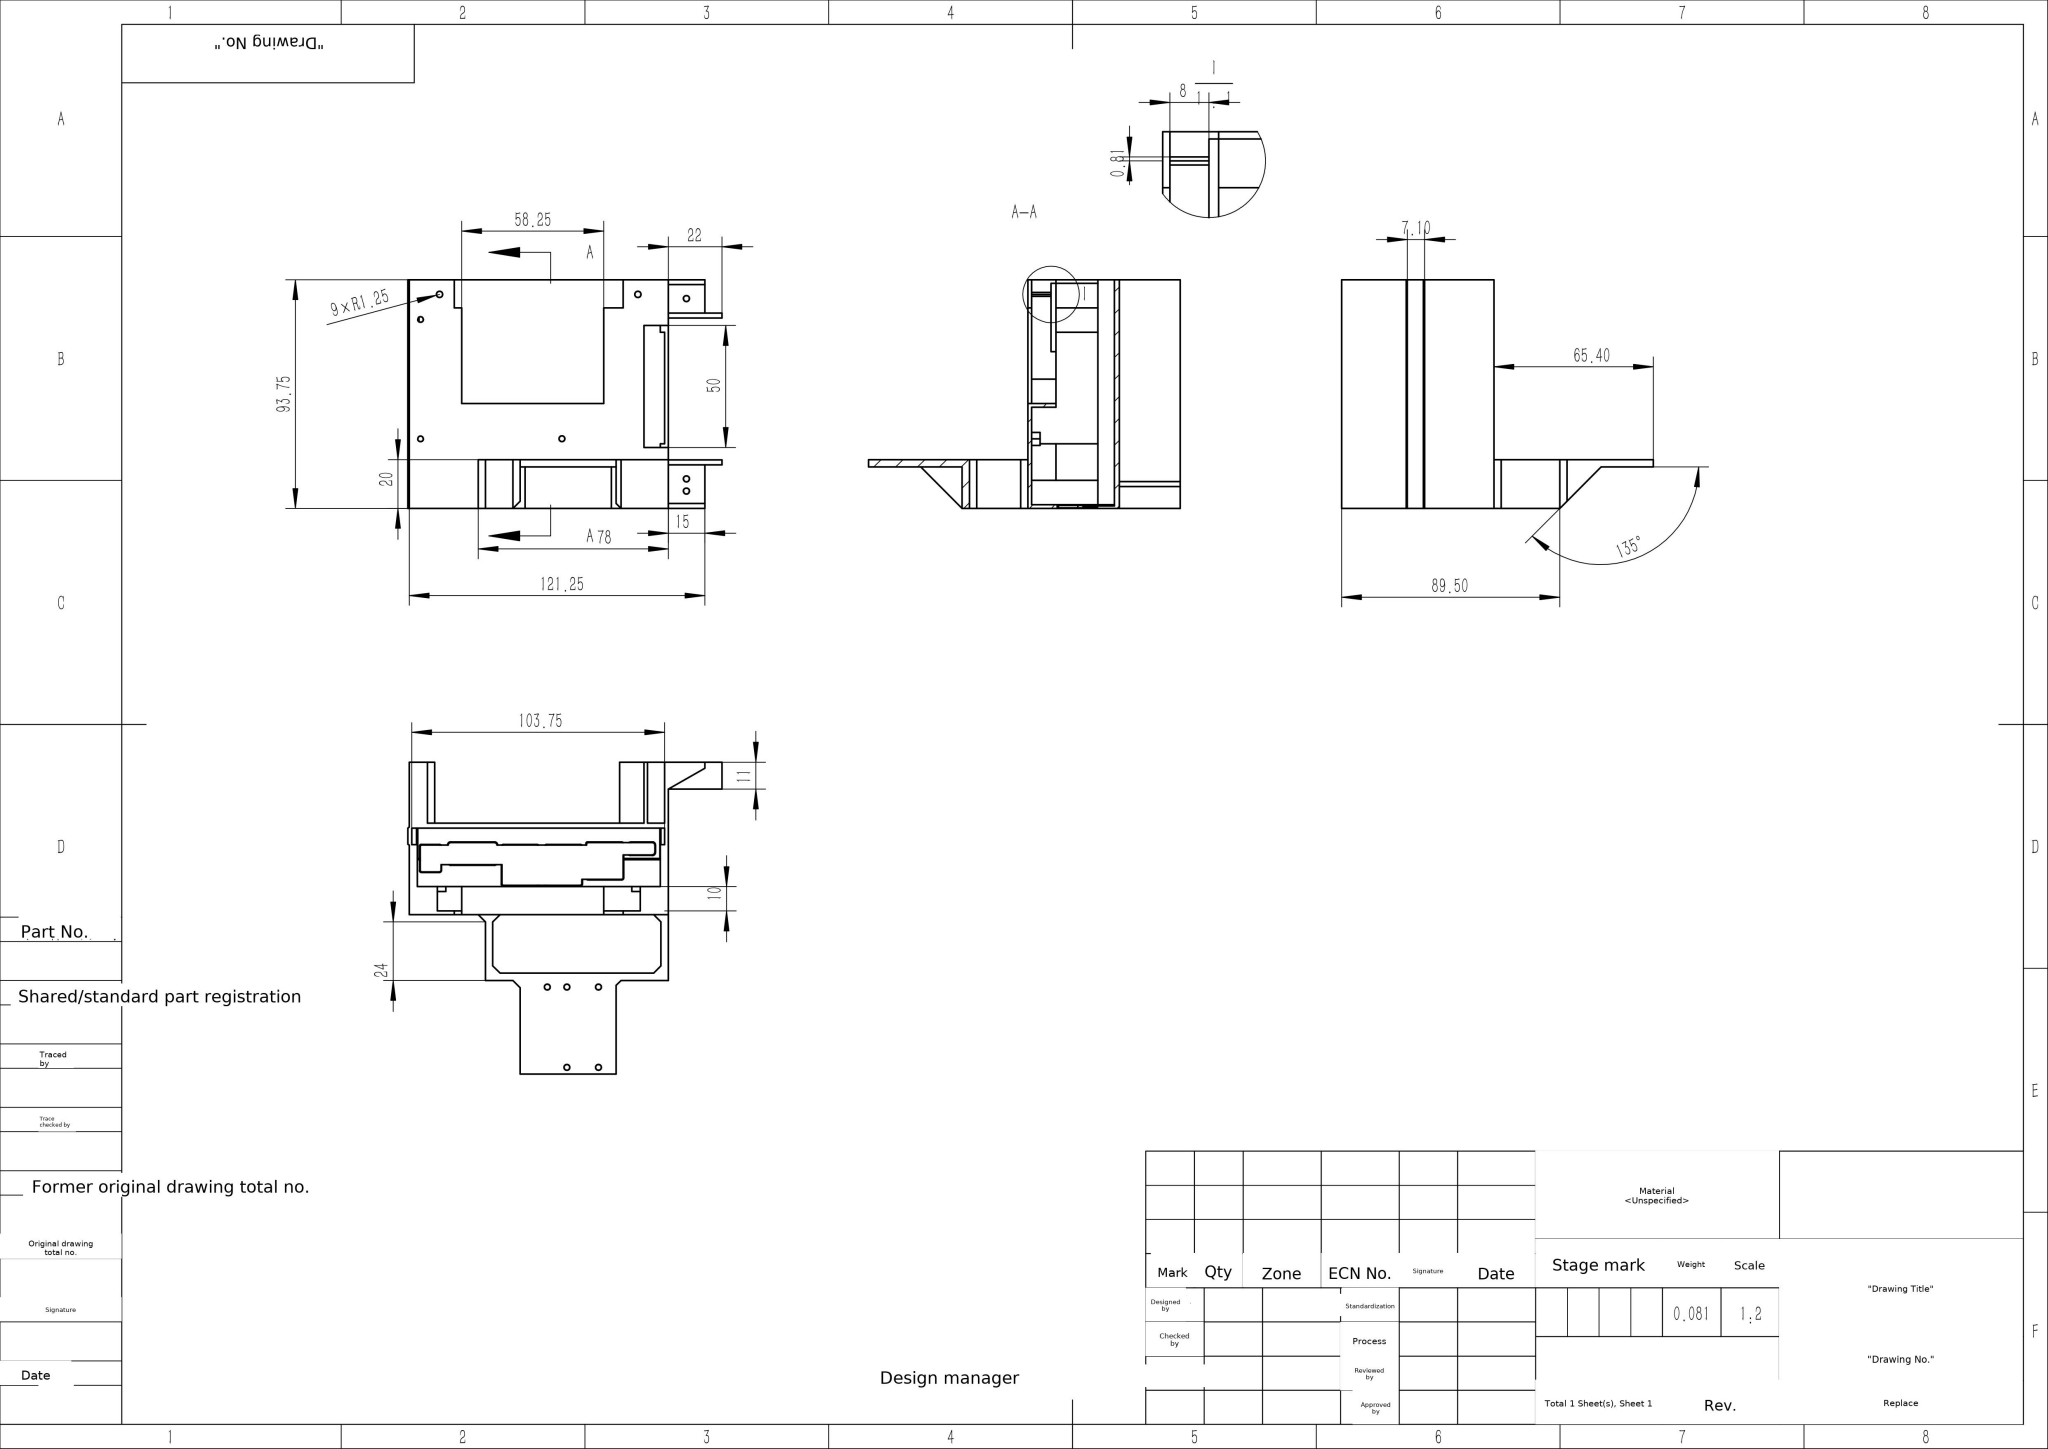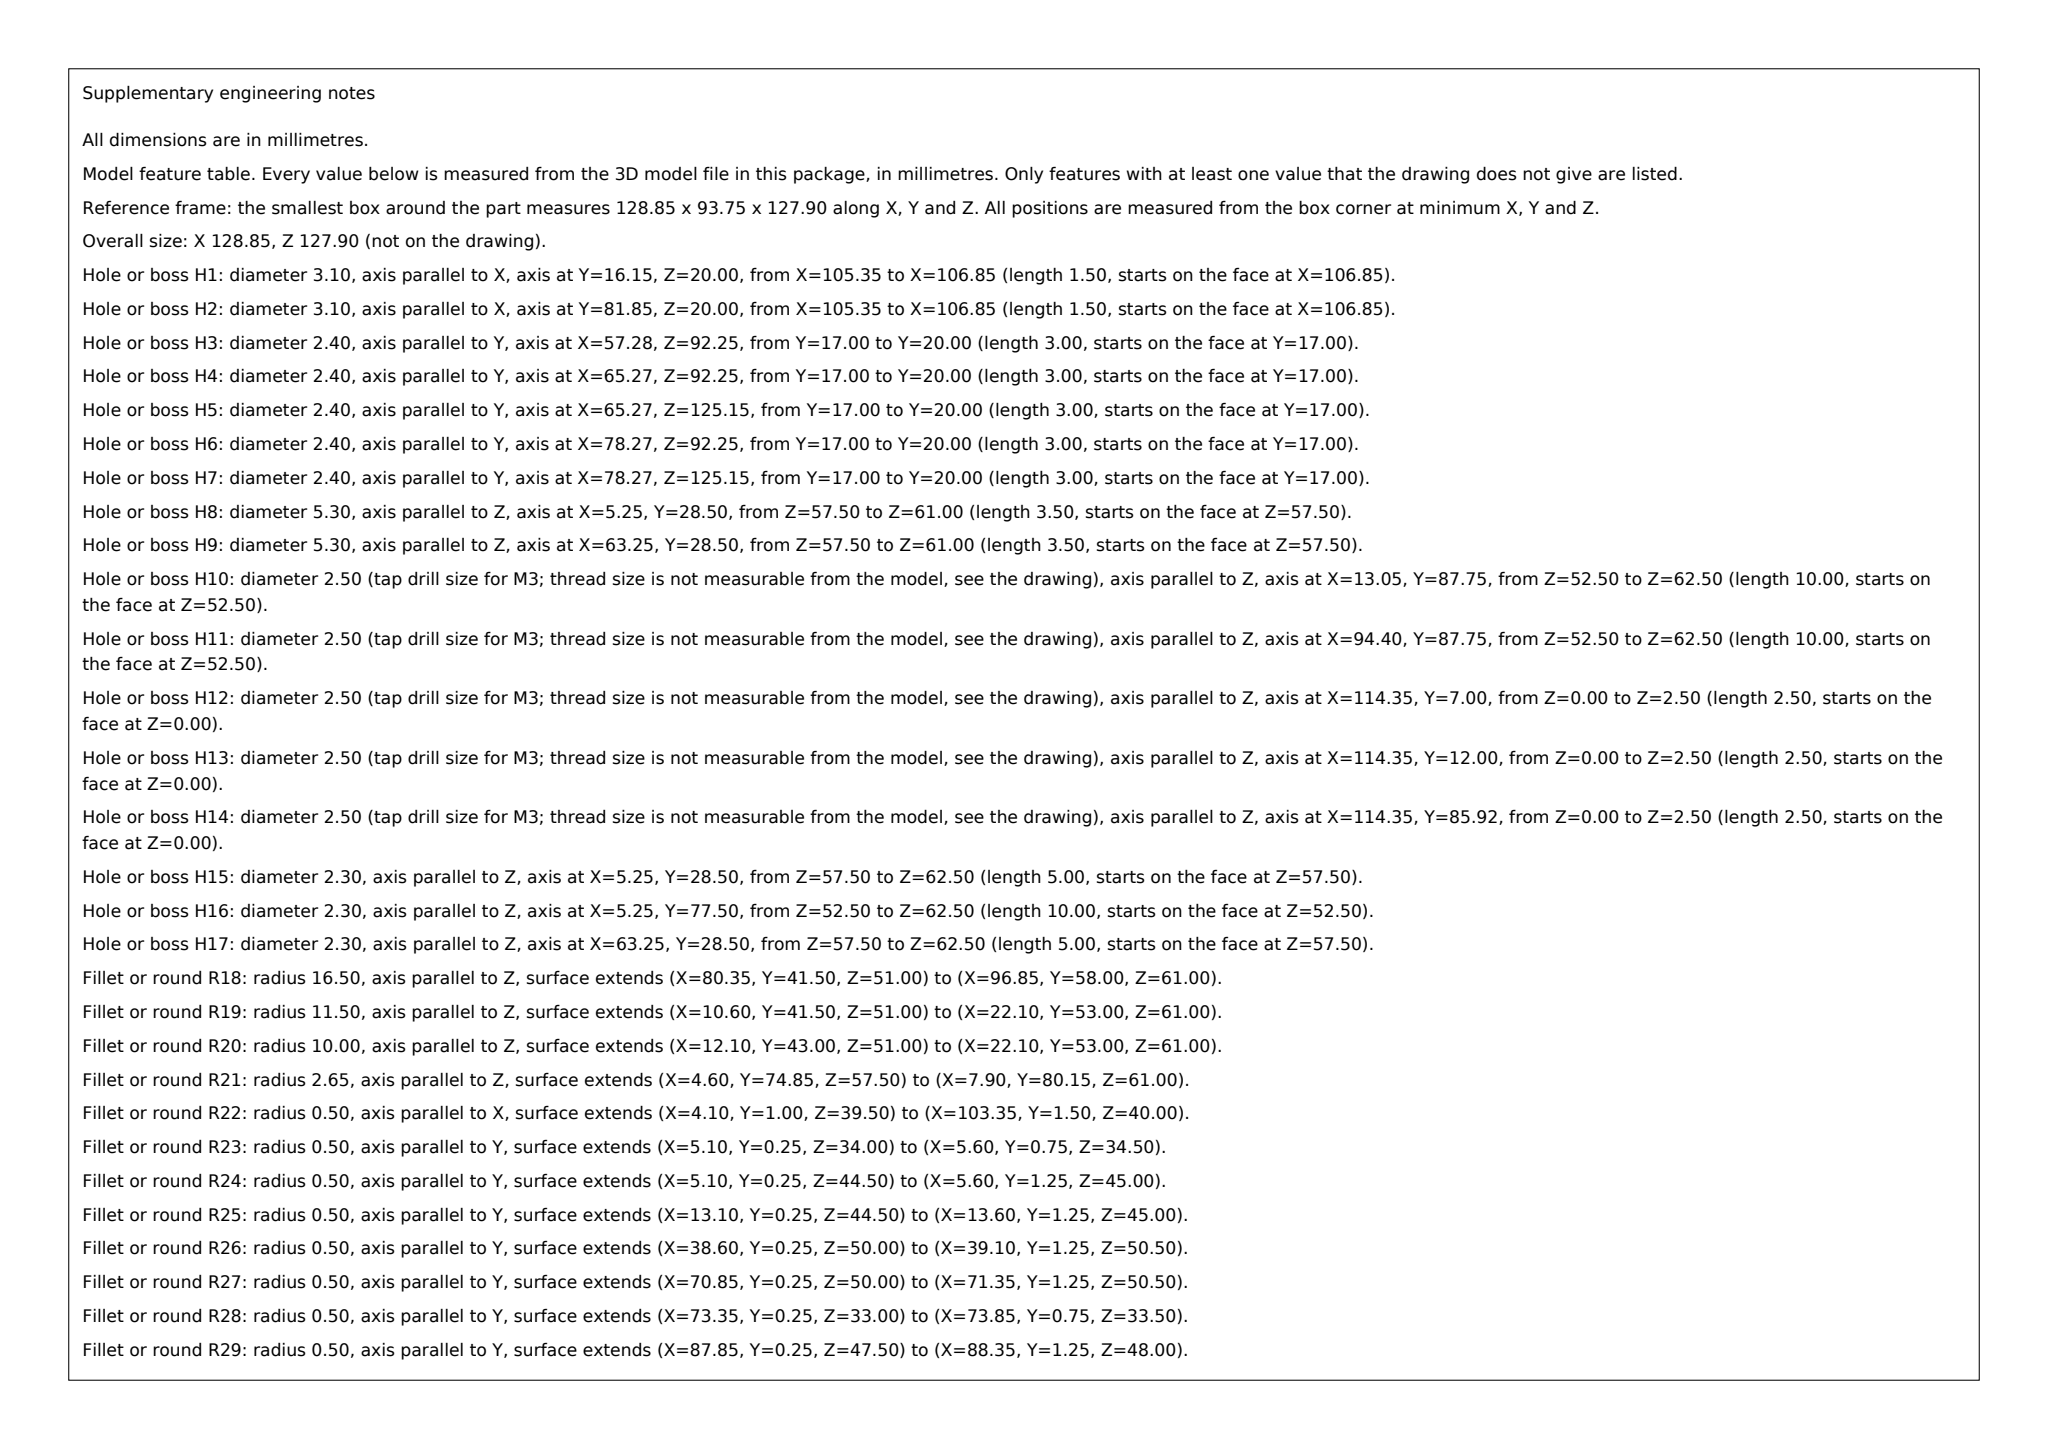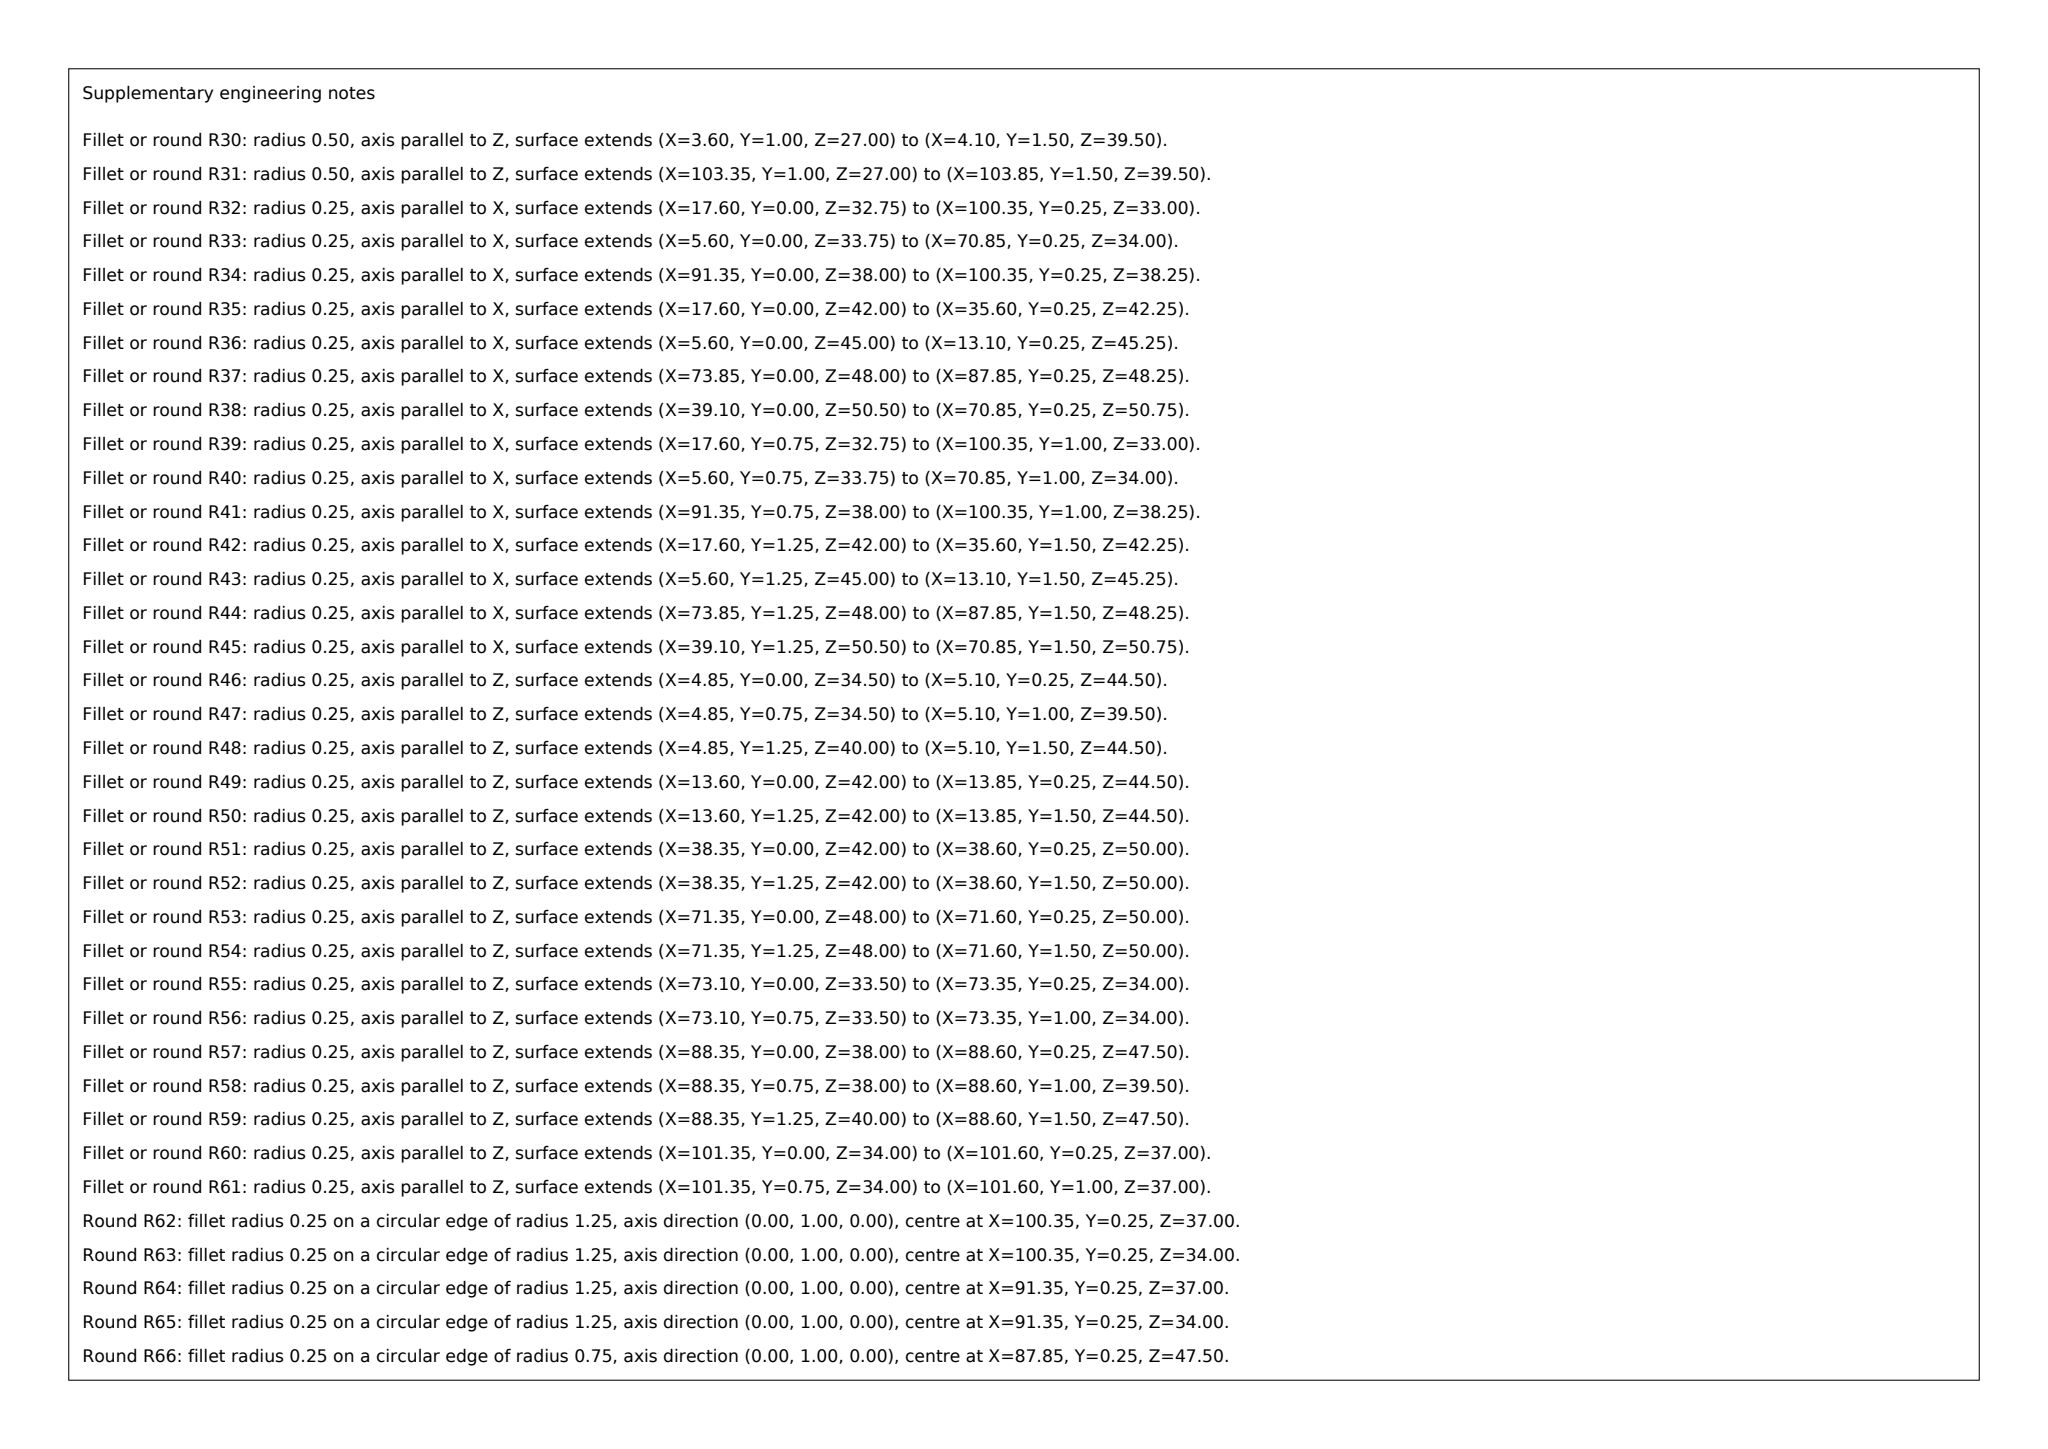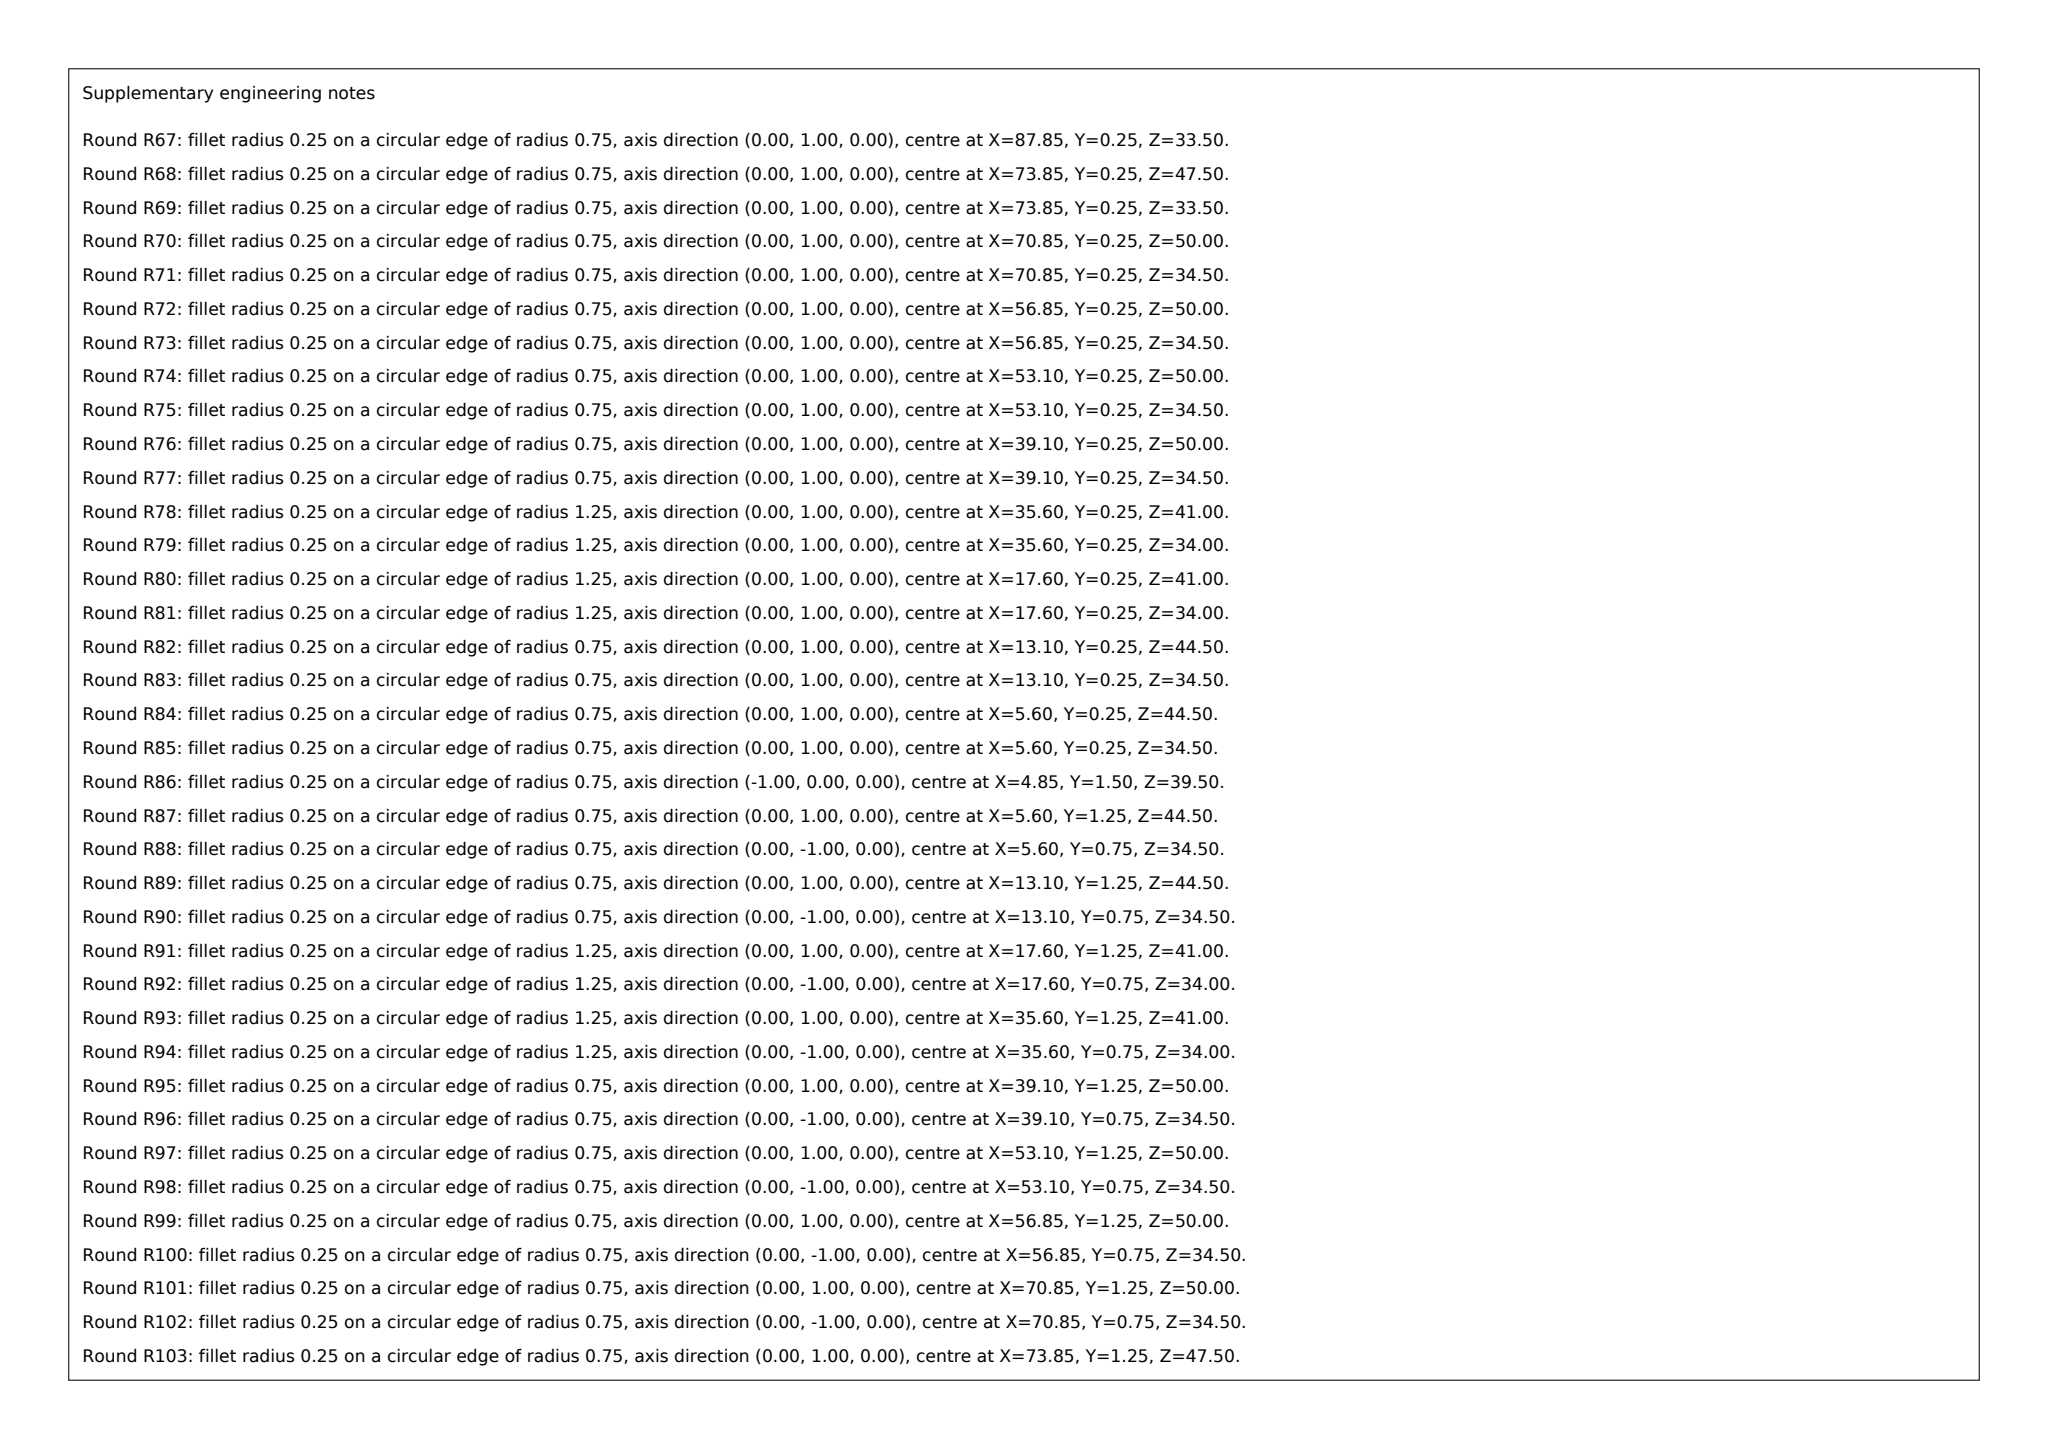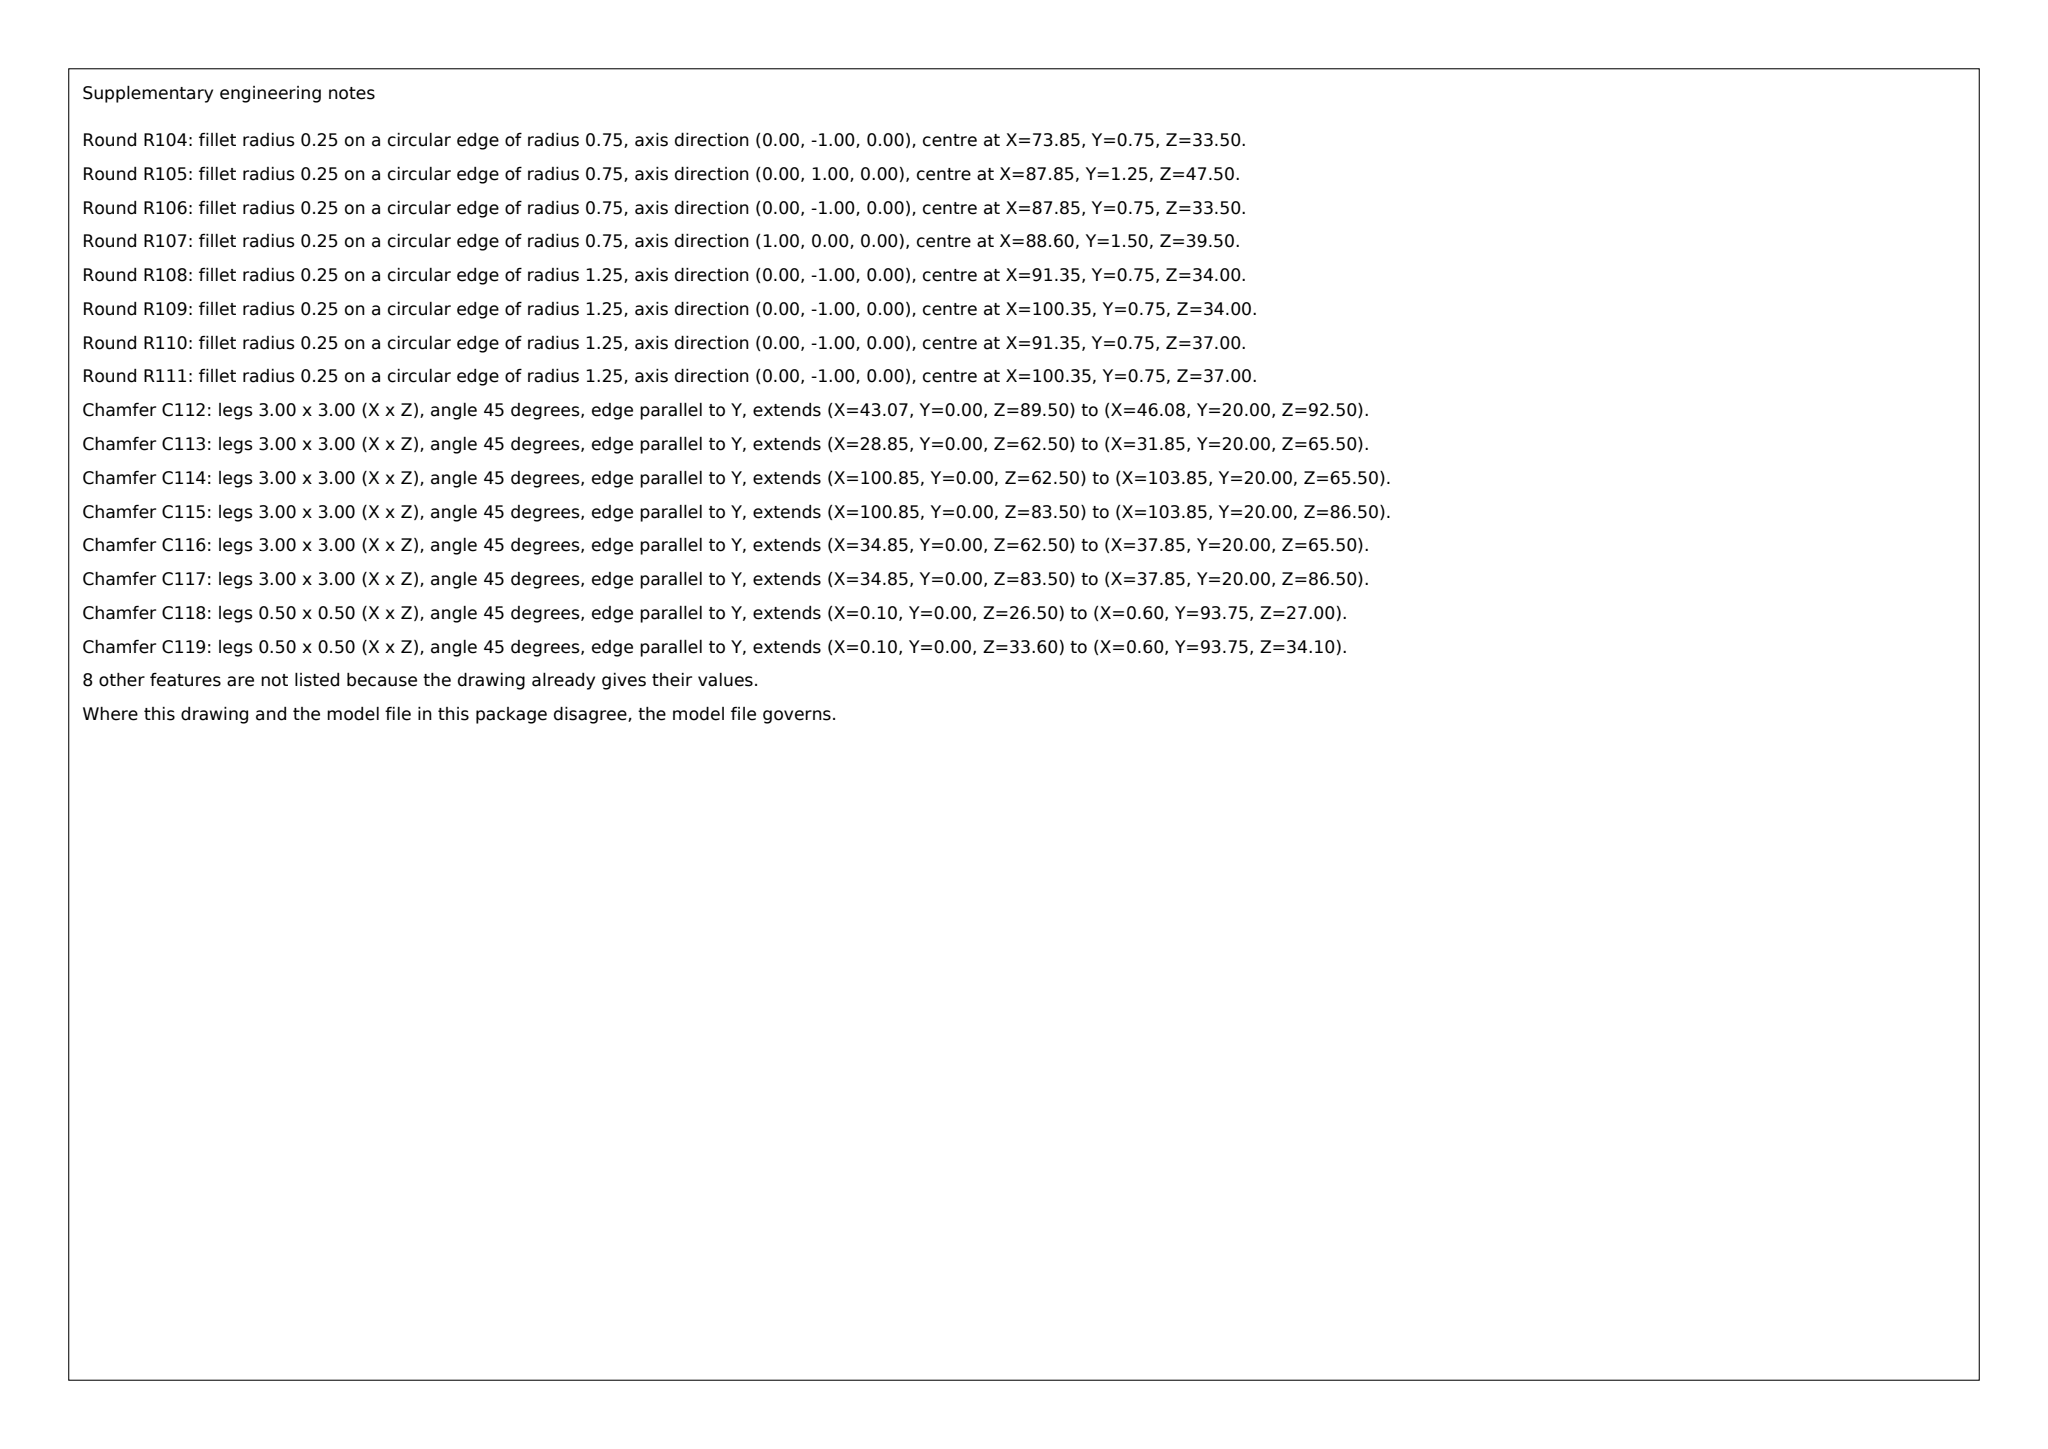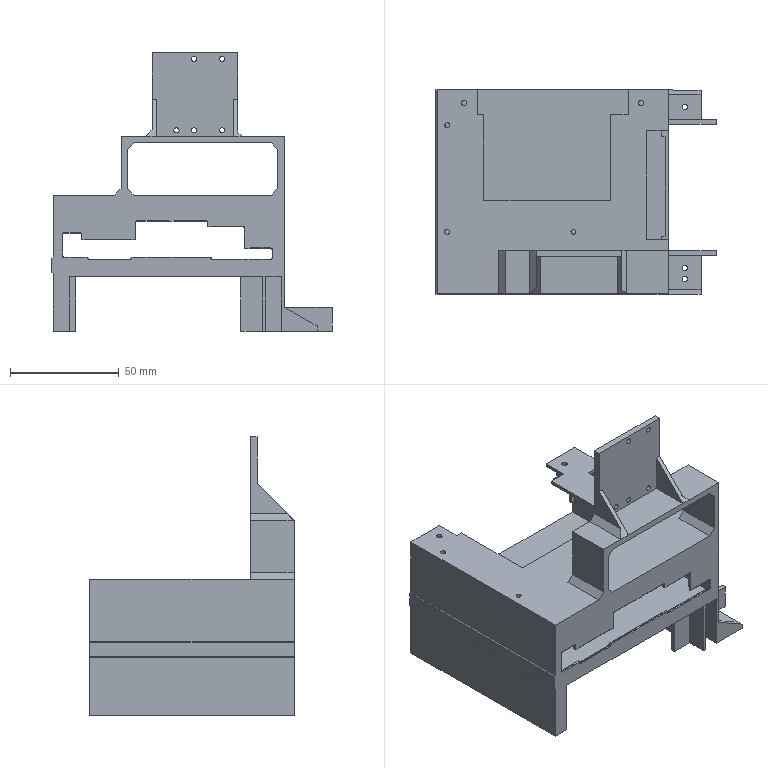Part | SolidWorks | mm | 1 solid | 344 faces | box 128.85 x 93.75 x 127.9 mm | volume 81459 mm3 | plane 196 | cylinder 96 | torus 50 | sphere 2 | commonest cylinder face diameters 0.5 x40 1 x11 2.5 x10 2.4 x10 5.3 x7 2.3 x6 3.1 x4 2 x4